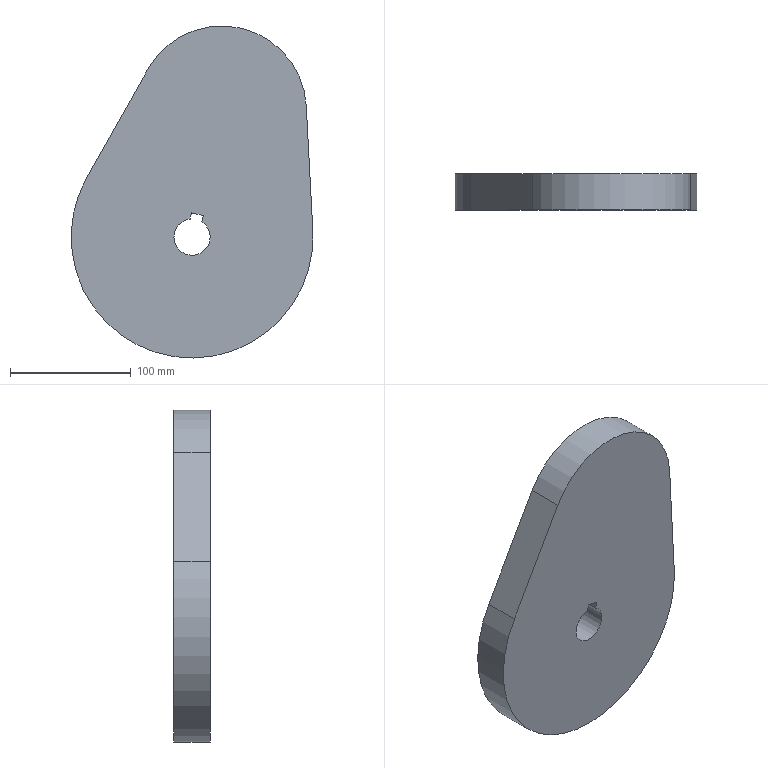Component | NX | CAM | 1 solid | 10 faces | box 200 x 30 x 274.65 mm | volume 1249246 mm3 | plane 7 | cylinder 3 | commonest cylinder face diameters 30 x1 200 x1 140 x1
STEP:
#1=CARTESIAN_POINT('',(0.,0.,0.));
#2=DIRECTION('',(0.,0.,1.));
#3=DIRECTION('',(1.,0.,0.));
#4=AXIS2_PLACEMENT_3D('',#1,#2,#3);
#5=CARTESIAN_POINT('',(298.366,15.,104.911));
#6=VERTEX_POINT('',#5);
#7=CARTESIAN_POINT('',(298.366,-15.,104.911));
#8=VERTEX_POINT('',#7);
#9=CARTESIAN_POINT('',(298.366,15.,104.911));
#10=DIRECTION('',(0.,-1.,0.));
#11=VECTOR('',#10,1.);
#12=LINE('',#9,#11);
#13=CARTESIAN_POINT('',(300.,15.,90.));
#14=DIRECTION('',(0.,-1.,0.));
#15=DIRECTION('',(-0.2286,0.,-0.9735));
#16=AXIS2_PLACEMENT_3D('',#13,#14,#15);
#17=CYLINDRICAL_SURFACE('',#16,15.);
#18=CARTESIAN_POINT('',(3.481,0.));
#19=DIRECTION('',(0.,1.));
#20=VECTOR('',#19,1.);
#21=LINE('',#18,#20);
#22=(GEOMETRIC_REPRESENTATION_CONTEXT(2)PARAMETRIC_REPRESENTATION_CONTEXT()REPRESENTATION_CONTEXT('',''));
#23=DEFINITIONAL_REPRESENTATION('',(#21),#22);
#24=PCURVE('',#17,#23);
#25=CARTESIAN_POINT('',(299.59,15.,110.127));
#26=DIRECTION('',(-0.9735,0.,0.2286));
#27=DIRECTION('',(0.2286,0.,0.9735));
#28=AXIS2_PLACEMENT_3D('',#25,#26,#27);
#29=PLANE('',#28);
#30=CARTESIAN_POINT('',(-5.358,0.));
#31=DIRECTION('',(0.,-1.));
#32=VECTOR('',#31,1.);
#33=LINE('',#30,#32);
#34=(GEOMETRIC_REPRESENTATION_CONTEXT(2)PARAMETRIC_REPRESENTATION_CONTEXT()REPRESENTATION_CONTEXT('',''));
#35=DEFINITIONAL_REPRESENTATION('',(#33),#34);
#36=PCURVE('',#29,#35);
#37=SURFACE_CURVE('',#12,(#24,#36),.PCURVE_S1.);
#38=EDGE_CURVE('',#6,#8,#37,.T.);
#39=ORIENTED_EDGE('',*,*,#38,.F.);
#40=CARTESIAN_POINT('',(308.101,15.,102.625));
#41=VERTEX_POINT('',#40);
#42=CARTESIAN_POINT('',(300.,15.,90.));
#43=DIRECTION('',(0.,-1.,0.));
#44=DIRECTION('',(0.2286,0.,0.9735));
#45=AXIS2_PLACEMENT_3D('',#42,#43,#44);
#46=CIRCLE('',#45,15.);
#47=CARTESIAN_POINT('',(3.142,0.));
#48=DIRECTION('',(1.,0.));
#49=VECTOR('',#48,1.);
#50=LINE('',#47,#49);
#51=(GEOMETRIC_REPRESENTATION_CONTEXT(2)PARAMETRIC_REPRESENTATION_CONTEXT()REPRESENTATION_CONTEXT('',''));
#52=DEFINITIONAL_REPRESENTATION('',(#50),#51);
#53=PCURVE('',#17,#52);
#54=CARTESIAN_POINT('',(300.,15.,90.));
#55=DIRECTION('',(0.,1.,0.));
#56=DIRECTION('',(0.2286,0.,0.9735));
#57=AXIS2_PLACEMENT_3D('',#54,#55,#56);
#58=PLANE('',#57);
#59=CARTESIAN_POINT('',(15.,0.));
#60=CARTESIAN_POINT('',(15.,-25.981));
#61=CARTESIAN_POINT('',(-7.5,-12.99));
#62=CARTESIAN_POINT('',(-30.,-0.));
#63=CARTESIAN_POINT('',(-7.5,12.99));
#64=CARTESIAN_POINT('',(15.,25.981));
#65=CARTESIAN_POINT('',(15.,0.));
#66=(BOUNDED_CURVE()B_SPLINE_CURVE(2,(#59,#60,#61,#62,#63,#64,#65),.UNSPECIFIED.,.T.,.F.)B_SPLINE_CURVE_WITH_KNOTS((1,2,2,2,2,1),(-2.094,0.,2.094,4.189,6.283,8.378),.UNSPECIFIED.)CURVE()GEOMETRIC_REPRESENTATION_ITEM()RATIONAL_B_SPLINE_CURVE((1.,0.5,1.,0.5,1.,0.5,1.))REPRESENTATION_ITEM(''));
#67=(GEOMETRIC_REPRESENTATION_CONTEXT(2)PARAMETRIC_REPRESENTATION_CONTEXT()REPRESENTATION_CONTEXT('',''));
#68=DEFINITIONAL_REPRESENTATION('',(#66),#67);
#69=PCURVE('',#58,#68);
#70=SURFACE_CURVE('',#46,(#53,#69),.PCURVE_S1.);
#71=EDGE_CURVE('',#6,#41,#70,.T.);
#72=ORIENTED_EDGE('',*,*,#71,.T.);
#73=CARTESIAN_POINT('',(308.101,-15.,102.625));
#74=VERTEX_POINT('',#73);
#75=CARTESIAN_POINT('',(308.101,15.,102.625));
#76=DIRECTION('',(0.,-1.,0.));
#77=VECTOR('',#76,1.);
#78=LINE('',#75,#77);
#79=CARTESIAN_POINT('',(9.085,0.));
#80=DIRECTION('',(0.,1.));
#81=VECTOR('',#80,1.);
#82=LINE('',#79,#81);
#83=(GEOMETRIC_REPRESENTATION_CONTEXT(2)PARAMETRIC_REPRESENTATION_CONTEXT()REPRESENTATION_CONTEXT('',''));
#84=DEFINITIONAL_REPRESENTATION('',(#82),#83);
#85=PCURVE('',#17,#84);
#86=CARTESIAN_POINT('',(308.101,15.,102.625));
#87=DIRECTION('',(0.9735,0.,-0.2286));
#88=DIRECTION('',(-0.2286,0.,-0.9735));
#89=AXIS2_PLACEMENT_3D('',#86,#87,#88);
#90=PLANE('',#89);
#91=CARTESIAN_POINT('',(-0.,0.));
#92=DIRECTION('',(0.,-1.));
#93=VECTOR('',#92,1.);
#94=LINE('',#91,#93);
#95=(GEOMETRIC_REPRESENTATION_CONTEXT(2)PARAMETRIC_REPRESENTATION_CONTEXT()REPRESENTATION_CONTEXT('',''));
#96=DEFINITIONAL_REPRESENTATION('',(#94),#95);
#97=PCURVE('',#90,#96);
#98=SURFACE_CURVE('',#78,(#85,#97),.PCURVE_S1.);
#99=EDGE_CURVE('',#41,#74,#98,.T.);
#100=ORIENTED_EDGE('',*,*,#99,.T.);
#101=CARTESIAN_POINT('',(300.,-15.,90.));
#102=DIRECTION('',(0.,-1.,0.));
#103=DIRECTION('',(0.2286,0.,0.9735));
#104=AXIS2_PLACEMENT_3D('',#101,#102,#103);
#105=CIRCLE('',#104,15.);
#106=CARTESIAN_POINT('',(3.142,30.));
#107=DIRECTION('',(1.,0.));
#108=VECTOR('',#107,1.);
#109=LINE('',#106,#108);
#110=(GEOMETRIC_REPRESENTATION_CONTEXT(2)PARAMETRIC_REPRESENTATION_CONTEXT()REPRESENTATION_CONTEXT('',''));
#111=DEFINITIONAL_REPRESENTATION('',(#109),#110);
#112=PCURVE('',#17,#111);
#113=CARTESIAN_POINT('',(300.,-15.,90.));
#114=DIRECTION('',(0.,1.,0.));
#115=DIRECTION('',(0.2286,0.,0.9735));
#116=AXIS2_PLACEMENT_3D('',#113,#114,#115);
#117=PLANE('',#116);
#118=CARTESIAN_POINT('',(15.,0.));
#119=CARTESIAN_POINT('',(15.,-25.981));
#120=CARTESIAN_POINT('',(-7.5,-12.99));
#121=CARTESIAN_POINT('',(-30.,-0.));
#122=CARTESIAN_POINT('',(-7.5,12.99));
#123=CARTESIAN_POINT('',(15.,25.981));
#124=CARTESIAN_POINT('',(15.,0.));
#125=(BOUNDED_CURVE()B_SPLINE_CURVE(2,(#118,#119,#120,#121,#122,#123,#124),.UNSPECIFIED.,.T.,.F.)B_SPLINE_CURVE_WITH_KNOTS((1,2,2,2,2,1),(-2.094,0.,2.094,4.189,6.283,8.378),.UNSPECIFIED.)CURVE()GEOMETRIC_REPRESENTATION_ITEM()RATIONAL_B_SPLINE_CURVE((1.,0.5,1.,0.5,1.,0.5,1.))REPRESENTATION_ITEM(''));
#126=(GEOMETRIC_REPRESENTATION_CONTEXT(2)PARAMETRIC_REPRESENTATION_CONTEXT()REPRESENTATION_CONTEXT('',''));
#127=DEFINITIONAL_REPRESENTATION('',(#125),#126);
#128=PCURVE('',#117,#127);
#129=SURFACE_CURVE('',#105,(#112,#128),.PCURVE_S1.);
#130=EDGE_CURVE('',#8,#74,#129,.T.);
#131=ORIENTED_EDGE('',*,*,#130,.F.);
#132=EDGE_LOOP('',(#39,#72,#100,#131));
#133=FACE_BOUND('',#132,.F.);
#134=ADVANCED_FACE('',(#133),#17,.F.);
#135=CARTESIAN_POINT('',(309.326,-15.,107.84));
#136=VERTEX_POINT('',#135);
#137=CARTESIAN_POINT('',(308.101,-15.,102.625));
#138=DIRECTION('',(0.2286,0.,0.9735));
#139=VECTOR('',#138,1.);
#140=LINE('',#137,#139);
#141=CARTESIAN_POINT('',(0.,-30.));
#142=DIRECTION('',(-1.,0.));
#143=VECTOR('',#142,1.);
#144=LINE('',#141,#143);
#145=(GEOMETRIC_REPRESENTATION_CONTEXT(2)PARAMETRIC_REPRESENTATION_CONTEXT()REPRESENTATION_CONTEXT('',''));
#146=DEFINITIONAL_REPRESENTATION('',(#144),#145);
#147=PCURVE('',#90,#146);
#148=CARTESIAN_POINT('',(14.142,5.));
#149=DIRECTION('',(1.,0.));
#150=VECTOR('',#149,1.);
#151=LINE('',#148,#150);
#152=(GEOMETRIC_REPRESENTATION_CONTEXT(2)PARAMETRIC_REPRESENTATION_CONTEXT()REPRESENTATION_CONTEXT('',''));
#153=DEFINITIONAL_REPRESENTATION('',(#151),#152);
#154=PCURVE('',#117,#153);
#155=SURFACE_CURVE('',#140,(#147,#154),.PCURVE_S1.);
#156=EDGE_CURVE('',#74,#136,#155,.T.);
#157=ORIENTED_EDGE('',*,*,#156,.T.);
#158=CARTESIAN_POINT('',(309.326,15.,107.84));
#159=VERTEX_POINT('',#158);
#160=CARTESIAN_POINT('',(309.326,15.,107.84));
#161=DIRECTION('',(0.,-1.,0.));
#162=VECTOR('',#161,1.);
#163=LINE('',#160,#162);
#164=CARTESIAN_POINT('',(-5.358,0.));
#165=DIRECTION('',(0.,-1.));
#166=VECTOR('',#165,1.);
#167=LINE('',#164,#166);
#168=(GEOMETRIC_REPRESENTATION_CONTEXT(2)PARAMETRIC_REPRESENTATION_CONTEXT()REPRESENTATION_CONTEXT('',''));
#169=DEFINITIONAL_REPRESENTATION('',(#167),#168);
#170=PCURVE('',#90,#169);
#171=CARTESIAN_POINT('',(309.326,15.,107.84));
#172=DIRECTION('',(0.2286,0.,0.9735));
#173=DIRECTION('',(0.9735,0.,-0.2286));
#174=AXIS2_PLACEMENT_3D('',#171,#172,#173);
#175=PLANE('',#174);
#176=CARTESIAN_POINT('',(0.,0.));
#177=DIRECTION('',(0.,-1.));
#178=VECTOR('',#177,1.);
#179=LINE('',#176,#178);
#180=(GEOMETRIC_REPRESENTATION_CONTEXT(2)PARAMETRIC_REPRESENTATION_CONTEXT()REPRESENTATION_CONTEXT('',''));
#181=DEFINITIONAL_REPRESENTATION('',(#179),#180);
#182=PCURVE('',#175,#181);
#183=SURFACE_CURVE('',#163,(#170,#182),.PCURVE_S1.);
#184=EDGE_CURVE('',#159,#136,#183,.T.);
#185=ORIENTED_EDGE('',*,*,#184,.F.);
#186=CARTESIAN_POINT('',(308.101,15.,102.625));
#187=DIRECTION('',(0.2286,0.,0.9735));
#188=VECTOR('',#187,1.);
#189=LINE('',#186,#188);
#190=CARTESIAN_POINT('',(0.,0.));
#191=DIRECTION('',(-1.,0.));
#192=VECTOR('',#191,1.);
#193=LINE('',#190,#192);
#194=(GEOMETRIC_REPRESENTATION_CONTEXT(2)PARAMETRIC_REPRESENTATION_CONTEXT()REPRESENTATION_CONTEXT('',''));
#195=DEFINITIONAL_REPRESENTATION('',(#193),#194);
#196=PCURVE('',#90,#195);
#197=CARTESIAN_POINT('',(14.142,5.));
#198=DIRECTION('',(1.,0.));
#199=VECTOR('',#198,1.);
#200=LINE('',#197,#199);
#201=(GEOMETRIC_REPRESENTATION_CONTEXT(2)PARAMETRIC_REPRESENTATION_CONTEXT()REPRESENTATION_CONTEXT('',''));
#202=DEFINITIONAL_REPRESENTATION('',(#200),#201);
#203=PCURVE('',#58,#202);
#204=SURFACE_CURVE('',#189,(#196,#203),.PCURVE_S1.);
#205=EDGE_CURVE('',#41,#159,#204,.T.);
#206=ORIENTED_EDGE('',*,*,#205,.F.);
#207=ORIENTED_EDGE('',*,*,#99,.T.);
#208=EDGE_LOOP('',(#157,#185,#206,#207));
#209=FACE_BOUND('',#208,.T.);
#210=ADVANCED_FACE('',(#209),#90,.F.);
#211=CARTESIAN_POINT('',(299.59,-15.,110.127));
#212=VERTEX_POINT('',#211);
#213=CARTESIAN_POINT('',(309.326,-15.,107.84));
#214=DIRECTION('',(-0.9735,0.,0.2286));
#215=VECTOR('',#214,1.);
#216=LINE('',#213,#215);
#217=CARTESIAN_POINT('',(0.,-30.));
#218=DIRECTION('',(-1.,0.));
#219=VECTOR('',#218,1.);
#220=LINE('',#217,#219);
#221=(GEOMETRIC_REPRESENTATION_CONTEXT(2)PARAMETRIC_REPRESENTATION_CONTEXT()REPRESENTATION_CONTEXT('',''));
#222=DEFINITIONAL_REPRESENTATION('',(#220),#221);
#223=PCURVE('',#175,#222);
#224=CARTESIAN_POINT('',(19.5,5.));
#225=DIRECTION('',(0.,-1.));
#226=VECTOR('',#225,1.);
#227=LINE('',#224,#226);
#228=(GEOMETRIC_REPRESENTATION_CONTEXT(2)PARAMETRIC_REPRESENTATION_CONTEXT()REPRESENTATION_CONTEXT('',''));
#229=DEFINITIONAL_REPRESENTATION('',(#227),#228);
#230=PCURVE('',#117,#229);
#231=SURFACE_CURVE('',#216,(#223,#230),.PCURVE_S1.);
#232=EDGE_CURVE('',#136,#212,#231,.T.);
#233=ORIENTED_EDGE('',*,*,#232,.T.);
#234=CARTESIAN_POINT('',(299.59,15.,110.127));
#235=VERTEX_POINT('',#234);
#236=CARTESIAN_POINT('',(299.59,15.,110.127));
#237=DIRECTION('',(0.,-1.,0.));
#238=VECTOR('',#237,1.);
#239=LINE('',#236,#238);
#240=CARTESIAN_POINT('',(-10.,0.));
#241=DIRECTION('',(0.,-1.));
#242=VECTOR('',#241,1.);
#243=LINE('',#240,#242);
#244=(GEOMETRIC_REPRESENTATION_CONTEXT(2)PARAMETRIC_REPRESENTATION_CONTEXT()REPRESENTATION_CONTEXT('',''));
#245=DEFINITIONAL_REPRESENTATION('',(#243),#244);
#246=PCURVE('',#175,#245);
#247=CARTESIAN_POINT('',(0.,0.));
#248=DIRECTION('',(0.,-1.));
#249=VECTOR('',#248,1.);
#250=LINE('',#247,#249);
#251=(GEOMETRIC_REPRESENTATION_CONTEXT(2)PARAMETRIC_REPRESENTATION_CONTEXT()REPRESENTATION_CONTEXT('',''));
#252=DEFINITIONAL_REPRESENTATION('',(#250),#251);
#253=PCURVE('',#29,#252);
#254=SURFACE_CURVE('',#239,(#246,#253),.PCURVE_S1.);
#255=EDGE_CURVE('',#235,#212,#254,.T.);
#256=ORIENTED_EDGE('',*,*,#255,.F.);
#257=CARTESIAN_POINT('',(309.326,15.,107.84));
#258=DIRECTION('',(-0.9735,0.,0.2286));
#259=VECTOR('',#258,1.);
#260=LINE('',#257,#259);
#261=CARTESIAN_POINT('',(0.,0.));
#262=DIRECTION('',(-1.,0.));
#263=VECTOR('',#262,1.);
#264=LINE('',#261,#263);
#265=(GEOMETRIC_REPRESENTATION_CONTEXT(2)PARAMETRIC_REPRESENTATION_CONTEXT()REPRESENTATION_CONTEXT('',''));
#266=DEFINITIONAL_REPRESENTATION('',(#264),#265);
#267=PCURVE('',#175,#266);
#268=CARTESIAN_POINT('',(19.5,5.));
#269=DIRECTION('',(0.,-1.));
#270=VECTOR('',#269,1.);
#271=LINE('',#268,#270);
#272=(GEOMETRIC_REPRESENTATION_CONTEXT(2)PARAMETRIC_REPRESENTATION_CONTEXT()REPRESENTATION_CONTEXT('',''));
#273=DEFINITIONAL_REPRESENTATION('',(#271),#272);
#274=PCURVE('',#58,#273);
#275=SURFACE_CURVE('',#260,(#267,#274),.PCURVE_S1.);
#276=EDGE_CURVE('',#159,#235,#275,.T.);
#277=ORIENTED_EDGE('',*,*,#276,.F.);
#278=ORIENTED_EDGE('',*,*,#184,.T.);
#279=EDGE_LOOP('',(#233,#256,#277,#278));
#280=FACE_BOUND('',#279,.T.);
#281=ADVANCED_FACE('',(#280),#175,.F.);
#282=CARTESIAN_POINT('',(399.864,-15.,95.214));
#283=VERTEX_POINT('',#282);
#284=CARTESIAN_POINT('',(212.896,-15.,139.121));
#285=VERTEX_POINT('',#284);
#286=CARTESIAN_POINT('',(300.,-15.,90.));
#287=DIRECTION('',(0.,1.,0.));
#288=DIRECTION('',(0.2286,0.,0.9735));
#289=AXIS2_PLACEMENT_3D('',#286,#287,#288);
#290=CIRCLE('',#289,100.);
#291=CARTESIAN_POINT('',(300.,15.,90.));
#292=DIRECTION('',(0.,-1.,0.));
#293=DIRECTION('',(-0.2286,0.,-0.9735));
#294=AXIS2_PLACEMENT_3D('',#291,#292,#293);
#295=CYLINDRICAL_SURFACE('',#294,100.);
#296=CARTESIAN_POINT('',(3.142,30.));
#297=DIRECTION('',(-1.,0.));
#298=VECTOR('',#297,1.);
#299=LINE('',#296,#298);
#300=(GEOMETRIC_REPRESENTATION_CONTEXT(2)PARAMETRIC_REPRESENTATION_CONTEXT()REPRESENTATION_CONTEXT('',''));
#301=DEFINITIONAL_REPRESENTATION('',(#299),#300);
#302=PCURVE('',#295,#301);
#303=CARTESIAN_POINT('',(0.,0.));
#304=DIRECTION('',(1.,0.));
#305=AXIS2_PLACEMENT_2D('',#303,#304);
#306=CIRCLE('',#305,100.);
#307=(GEOMETRIC_REPRESENTATION_CONTEXT(2)PARAMETRIC_REPRESENTATION_CONTEXT()REPRESENTATION_CONTEXT('',''));
#308=DEFINITIONAL_REPRESENTATION('',(#306),#307);
#309=PCURVE('',#117,#308);
#310=SURFACE_CURVE('',#290,(#302,#309),.PCURVE_S1.);
#311=EDGE_CURVE('',#283,#285,#310,.T.);
#312=ORIENTED_EDGE('',*,*,#311,.T.);
#313=CARTESIAN_POINT('',(212.896,15.,139.121));
#314=VERTEX_POINT('',#313);
#315=CARTESIAN_POINT('',(212.896,15.,139.121));
#316=DIRECTION('',(0.,-1.,0.));
#317=VECTOR('',#316,1.);
#318=LINE('',#315,#317);
#319=CARTESIAN_POINT('',(-1.854,0.));
#320=DIRECTION('',(0.,1.));
#321=VECTOR('',#320,1.);
#322=LINE('',#319,#321);
#323=(GEOMETRIC_REPRESENTATION_CONTEXT(2)PARAMETRIC_REPRESENTATION_CONTEXT()REPRESENTATION_CONTEXT('',''));
#324=DEFINITIONAL_REPRESENTATION('',(#322),#323);
#325=PCURVE('',#295,#324);
#326=CARTESIAN_POINT('',(212.896,15.,139.121));
#327=DIRECTION('',(0.871,0.,-0.4912));
#328=DIRECTION('',(-0.4912,0.,-0.871));
#329=AXIS2_PLACEMENT_3D('',#326,#327,#328);
#330=PLANE('',#329);
#331=CARTESIAN_POINT('',(0.,0.));
#332=DIRECTION('',(0.,-1.));
#333=VECTOR('',#332,1.);
#334=LINE('',#331,#333);
#335=(GEOMETRIC_REPRESENTATION_CONTEXT(2)PARAMETRIC_REPRESENTATION_CONTEXT()REPRESENTATION_CONTEXT('',''));
#336=DEFINITIONAL_REPRESENTATION('',(#334),#335);
#337=PCURVE('',#330,#336);
#338=SURFACE_CURVE('',#318,(#325,#337),.PCURVE_S1.);
#339=EDGE_CURVE('',#314,#285,#338,.T.);
#340=ORIENTED_EDGE('',*,*,#339,.F.);
#341=CARTESIAN_POINT('',(399.864,15.,95.214));
#342=VERTEX_POINT('',#341);
#343=CARTESIAN_POINT('',(300.,15.,90.));
#344=DIRECTION('',(0.,1.,0.));
#345=DIRECTION('',(0.2286,0.,0.9735));
#346=AXIS2_PLACEMENT_3D('',#343,#344,#345);
#347=CIRCLE('',#346,100.);
#348=CARTESIAN_POINT('',(3.142,0.));
#349=DIRECTION('',(-1.,0.));
#350=VECTOR('',#349,1.);
#351=LINE('',#348,#350);
#352=(GEOMETRIC_REPRESENTATION_CONTEXT(2)PARAMETRIC_REPRESENTATION_CONTEXT()REPRESENTATION_CONTEXT('',''));
#353=DEFINITIONAL_REPRESENTATION('',(#351),#352);
#354=PCURVE('',#295,#353);
#355=CARTESIAN_POINT('',(0.,0.));
#356=DIRECTION('',(1.,0.));
#357=AXIS2_PLACEMENT_2D('',#355,#356);
#358=CIRCLE('',#357,100.);
#359=(GEOMETRIC_REPRESENTATION_CONTEXT(2)PARAMETRIC_REPRESENTATION_CONTEXT()REPRESENTATION_CONTEXT('',''));
#360=DEFINITIONAL_REPRESENTATION('',(#358),#359);
#361=PCURVE('',#58,#360);
#362=SURFACE_CURVE('',#347,(#354,#361),.PCURVE_S1.);
#363=EDGE_CURVE('',#342,#314,#362,.T.);
#364=ORIENTED_EDGE('',*,*,#363,.F.);
#365=CARTESIAN_POINT('',(399.864,15.,95.214));
#366=DIRECTION('',(0.,-1.,0.));
#367=VECTOR('',#366,1.);
#368=LINE('',#365,#367);
#369=CARTESIAN_POINT('',(1.854,0.));
#370=DIRECTION('',(0.,1.));
#371=VECTOR('',#370,1.);
#372=LINE('',#369,#371);
#373=(GEOMETRIC_REPRESENTATION_CONTEXT(2)PARAMETRIC_REPRESENTATION_CONTEXT()REPRESENTATION_CONTEXT('',''));
#374=DEFINITIONAL_REPRESENTATION('',(#372),#373);
#375=PCURVE('',#295,#374);
#376=CARTESIAN_POINT('',(394.481,15.,198.303));
#377=DIRECTION('',(-0.9986,0.,-0.05214));
#378=DIRECTION('',(-0.05214,0.,0.9986));
#379=AXIS2_PLACEMENT_3D('',#376,#377,#378);
#380=PLANE('',#379);
#381=CARTESIAN_POINT('',(-103.229,0.));
#382=DIRECTION('',(0.,-1.));
#383=VECTOR('',#382,1.);
#384=LINE('',#381,#383);
#385=(GEOMETRIC_REPRESENTATION_CONTEXT(2)PARAMETRIC_REPRESENTATION_CONTEXT()REPRESENTATION_CONTEXT('',''));
#386=DEFINITIONAL_REPRESENTATION('',(#384),#385);
#387=PCURVE('',#380,#386);
#388=SURFACE_CURVE('',#368,(#375,#387),.PCURVE_S1.);
#389=EDGE_CURVE('',#342,#283,#388,.T.);
#390=ORIENTED_EDGE('',*,*,#389,.T.);
#391=EDGE_LOOP('',(#312,#340,#364,#390));
#392=FACE_BOUND('',#391,.T.);
#393=ADVANCED_FACE('',(#392),#295,.T.);
#394=CARTESIAN_POINT('',(263.604,-15.,229.038));
#395=VERTEX_POINT('',#394);
#396=CARTESIAN_POINT('',(212.896,-15.,139.121));
#397=DIRECTION('',(0.4912,0.,0.871));
#398=VECTOR('',#397,1.);
#399=LINE('',#396,#398);
#400=CARTESIAN_POINT('',(0.,-30.));
#401=DIRECTION('',(-1.,0.));
#402=VECTOR('',#401,1.);
#403=LINE('',#400,#402);
#404=(GEOMETRIC_REPRESENTATION_CONTEXT(2)PARAMETRIC_REPRESENTATION_CONTEXT()REPRESENTATION_CONTEXT('',''));
#405=DEFINITIONAL_REPRESENTATION('',(#403),#404);
#406=PCURVE('',#330,#405);
#407=CARTESIAN_POINT('',(27.907,-96.027));
#408=DIRECTION('',(0.9603,0.2791));
#409=VECTOR('',#408,1.);
#410=LINE('',#407,#409);
#411=(GEOMETRIC_REPRESENTATION_CONTEXT(2)PARAMETRIC_REPRESENTATION_CONTEXT()REPRESENTATION_CONTEXT('',''));
#412=DEFINITIONAL_REPRESENTATION('',(#410),#411);
#413=PCURVE('',#117,#412);
#414=SURFACE_CURVE('',#399,(#406,#413),.PCURVE_S1.);
#415=EDGE_CURVE('',#285,#395,#414,.T.);
#416=ORIENTED_EDGE('',*,*,#415,.T.);
#417=CARTESIAN_POINT('',(263.604,15.,229.038));
#418=VERTEX_POINT('',#417);
#419=CARTESIAN_POINT('',(263.604,15.,229.038));
#420=DIRECTION('',(0.,-1.,0.));
#421=VECTOR('',#420,1.);
#422=LINE('',#419,#421);
#423=CARTESIAN_POINT('',(-103.229,0.));
#424=DIRECTION('',(0.,-1.));
#425=VECTOR('',#424,1.);
#426=LINE('',#423,#425);
#427=(GEOMETRIC_REPRESENTATION_CONTEXT(2)PARAMETRIC_REPRESENTATION_CONTEXT()REPRESENTATION_CONTEXT('',''));
#428=DEFINITIONAL_REPRESENTATION('',(#426),#427);
#429=PCURVE('',#330,#428);
#430=CARTESIAN_POINT('',(324.576,15.,194.653));
#431=DIRECTION('',(0.,-1.,0.));
#432=DIRECTION('',(-0.2286,0.,-0.9735));
#433=AXIS2_PLACEMENT_3D('',#430,#431,#432);
#434=CYLINDRICAL_SURFACE('',#433,70.);
#435=CARTESIAN_POINT('',(4.43,0.));
#436=DIRECTION('',(0.,1.));
#437=VECTOR('',#436,1.);
#438=LINE('',#435,#437);
#439=(GEOMETRIC_REPRESENTATION_CONTEXT(2)PARAMETRIC_REPRESENTATION_CONTEXT()REPRESENTATION_CONTEXT('',''));
#440=DEFINITIONAL_REPRESENTATION('',(#438),#439);
#441=PCURVE('',#434,#440);
#442=SURFACE_CURVE('',#422,(#429,#441),.PCURVE_S1.);
#443=EDGE_CURVE('',#418,#395,#442,.T.);
#444=ORIENTED_EDGE('',*,*,#443,.F.);
#445=CARTESIAN_POINT('',(212.896,15.,139.121));
#446=DIRECTION('',(0.4912,0.,0.871));
#447=VECTOR('',#446,1.);
#448=LINE('',#445,#447);
#449=CARTESIAN_POINT('',(0.,0.));
#450=DIRECTION('',(-1.,0.));
#451=VECTOR('',#450,1.);
#452=LINE('',#449,#451);
#453=(GEOMETRIC_REPRESENTATION_CONTEXT(2)PARAMETRIC_REPRESENTATION_CONTEXT()REPRESENTATION_CONTEXT('',''));
#454=DEFINITIONAL_REPRESENTATION('',(#452),#453);
#455=PCURVE('',#330,#454);
#456=CARTESIAN_POINT('',(27.907,-96.027));
#457=DIRECTION('',(0.9603,0.2791));
#458=VECTOR('',#457,1.);
#459=LINE('',#456,#458);
#460=(GEOMETRIC_REPRESENTATION_CONTEXT(2)PARAMETRIC_REPRESENTATION_CONTEXT()REPRESENTATION_CONTEXT('',''));
#461=DEFINITIONAL_REPRESENTATION('',(#459),#460);
#462=PCURVE('',#58,#461);
#463=SURFACE_CURVE('',#448,(#455,#462),.PCURVE_S1.);
#464=EDGE_CURVE('',#314,#418,#463,.T.);
#465=ORIENTED_EDGE('',*,*,#464,.F.);
#466=ORIENTED_EDGE('',*,*,#339,.T.);
#467=EDGE_LOOP('',(#416,#444,#465,#466));
#468=FACE_BOUND('',#467,.T.);
#469=ADVANCED_FACE('',(#468),#330,.F.);
#470=CARTESIAN_POINT('',(394.481,-15.,198.303));
#471=VERTEX_POINT('',#470);
#472=CARTESIAN_POINT('',(324.576,-15.,194.653));
#473=DIRECTION('',(0.,1.,0.));
#474=DIRECTION('',(0.2286,0.,0.9735));
#475=AXIS2_PLACEMENT_3D('',#472,#473,#474);
#476=CIRCLE('',#475,70.);
#477=CARTESIAN_POINT('',(9.425,30.));
#478=DIRECTION('',(-1.,0.));
#479=VECTOR('',#478,1.);
#480=LINE('',#477,#479);
#481=(GEOMETRIC_REPRESENTATION_CONTEXT(2)PARAMETRIC_REPRESENTATION_CONTEXT()REPRESENTATION_CONTEXT('',''));
#482=DEFINITIONAL_REPRESENTATION('',(#480),#481);
#483=PCURVE('',#434,#482);
#484=CARTESIAN_POINT('',(107.5,0.));
#485=DIRECTION('',(1.,0.));
#486=AXIS2_PLACEMENT_2D('',#484,#485);
#487=CIRCLE('',#486,70.);
#488=(GEOMETRIC_REPRESENTATION_CONTEXT(2)PARAMETRIC_REPRESENTATION_CONTEXT()REPRESENTATION_CONTEXT('',''));
#489=DEFINITIONAL_REPRESENTATION('',(#487),#488);
#490=PCURVE('',#117,#489);
#491=SURFACE_CURVE('',#476,(#483,#490),.PCURVE_S1.);
#492=EDGE_CURVE('',#395,#471,#491,.T.);
#493=ORIENTED_EDGE('',*,*,#492,.T.);
#494=CARTESIAN_POINT('',(394.481,15.,198.303));
#495=VERTEX_POINT('',#494);
#496=CARTESIAN_POINT('',(394.481,15.,198.303));
#497=DIRECTION('',(0.,-1.,0.));
#498=VECTOR('',#497,1.);
#499=LINE('',#496,#498);
#500=CARTESIAN_POINT('',(1.854,0.));
#501=DIRECTION('',(0.,1.));
#502=VECTOR('',#501,1.);
#503=LINE('',#500,#502);
#504=(GEOMETRIC_REPRESENTATION_CONTEXT(2)PARAMETRIC_REPRESENTATION_CONTEXT()REPRESENTATION_CONTEXT('',''));
#505=DEFINITIONAL_REPRESENTATION('',(#503),#504);
#506=PCURVE('',#434,#505);
#507=CARTESIAN_POINT('',(0.,0.));
#508=DIRECTION('',(0.,-1.));
#509=VECTOR('',#508,1.);
#510=LINE('',#507,#509);
#511=(GEOMETRIC_REPRESENTATION_CONTEXT(2)PARAMETRIC_REPRESENTATION_CONTEXT()REPRESENTATION_CONTEXT('',''));
#512=DEFINITIONAL_REPRESENTATION('',(#510),#511);
#513=PCURVE('',#380,#512);
#514=SURFACE_CURVE('',#499,(#506,#513),.PCURVE_S1.);
#515=EDGE_CURVE('',#495,#471,#514,.T.);
#516=ORIENTED_EDGE('',*,*,#515,.F.);
#517=CARTESIAN_POINT('',(324.576,15.,194.653));
#518=DIRECTION('',(0.,1.,0.));
#519=DIRECTION('',(0.2286,0.,0.9735));
#520=AXIS2_PLACEMENT_3D('',#517,#518,#519);
#521=CIRCLE('',#520,70.);
#522=CARTESIAN_POINT('',(9.425,0.));
#523=DIRECTION('',(-1.,0.));
#524=VECTOR('',#523,1.);
#525=LINE('',#522,#524);
#526=(GEOMETRIC_REPRESENTATION_CONTEXT(2)PARAMETRIC_REPRESENTATION_CONTEXT()REPRESENTATION_CONTEXT('',''));
#527=DEFINITIONAL_REPRESENTATION('',(#525),#526);
#528=PCURVE('',#434,#527);
#529=CARTESIAN_POINT('',(107.5,0.));
#530=DIRECTION('',(1.,0.));
#531=AXIS2_PLACEMENT_2D('',#529,#530);
#532=CIRCLE('',#531,70.);
#533=(GEOMETRIC_REPRESENTATION_CONTEXT(2)PARAMETRIC_REPRESENTATION_CONTEXT()REPRESENTATION_CONTEXT('',''));
#534=DEFINITIONAL_REPRESENTATION('',(#532),#533);
#535=PCURVE('',#58,#534);
#536=SURFACE_CURVE('',#521,(#528,#535),.PCURVE_S1.);
#537=EDGE_CURVE('',#418,#495,#536,.T.);
#538=ORIENTED_EDGE('',*,*,#537,.F.);
#539=ORIENTED_EDGE('',*,*,#443,.T.);
#540=EDGE_LOOP('',(#493,#516,#538,#539));
#541=FACE_BOUND('',#540,.T.);
#542=ADVANCED_FACE('',(#541),#434,.T.);
#543=CARTESIAN_POINT('',(394.481,-15.,198.303));
#544=DIRECTION('',(0.05214,0.,-0.9986));
#545=VECTOR('',#544,1.);
#546=LINE('',#543,#545);
#547=CARTESIAN_POINT('',(0.,-30.));
#548=DIRECTION('',(-1.,0.));
#549=VECTOR('',#548,1.);
#550=LINE('',#547,#549);
#551=(GEOMETRIC_REPRESENTATION_CONTEXT(2)PARAMETRIC_REPRESENTATION_CONTEXT()REPRESENTATION_CONTEXT('',''));
#552=DEFINITIONAL_REPRESENTATION('',(#550),#551);
#553=PCURVE('',#380,#552);
#554=CARTESIAN_POINT('',(127.035,67.219));
#555=DIRECTION('',(-0.9603,0.2791));
#556=VECTOR('',#555,1.);
#557=LINE('',#554,#556);
#558=(GEOMETRIC_REPRESENTATION_CONTEXT(2)PARAMETRIC_REPRESENTATION_CONTEXT()REPRESENTATION_CONTEXT('',''));
#559=DEFINITIONAL_REPRESENTATION('',(#557),#558);
#560=PCURVE('',#117,#559);
#561=SURFACE_CURVE('',#546,(#553,#560),.PCURVE_S1.);
#562=EDGE_CURVE('',#471,#283,#561,.T.);
#563=ORIENTED_EDGE('',*,*,#562,.T.);
#564=ORIENTED_EDGE('',*,*,#389,.F.);
#565=CARTESIAN_POINT('',(394.481,15.,198.303));
#566=DIRECTION('',(0.05214,0.,-0.9986));
#567=VECTOR('',#566,1.);
#568=LINE('',#565,#567);
#569=CARTESIAN_POINT('',(0.,0.));
#570=DIRECTION('',(-1.,0.));
#571=VECTOR('',#570,1.);
#572=LINE('',#569,#571);
#573=(GEOMETRIC_REPRESENTATION_CONTEXT(2)PARAMETRIC_REPRESENTATION_CONTEXT()REPRESENTATION_CONTEXT('',''));
#574=DEFINITIONAL_REPRESENTATION('',(#572),#573);
#575=PCURVE('',#380,#574);
#576=CARTESIAN_POINT('',(127.035,67.219));
#577=DIRECTION('',(-0.9603,0.2791));
#578=VECTOR('',#577,1.);
#579=LINE('',#576,#578);
#580=(GEOMETRIC_REPRESENTATION_CONTEXT(2)PARAMETRIC_REPRESENTATION_CONTEXT()REPRESENTATION_CONTEXT('',''));
#581=DEFINITIONAL_REPRESENTATION('',(#579),#580);
#582=PCURVE('',#58,#581);
#583=SURFACE_CURVE('',#568,(#575,#582),.PCURVE_S1.);
#584=EDGE_CURVE('',#495,#342,#583,.T.);
#585=ORIENTED_EDGE('',*,*,#584,.F.);
#586=ORIENTED_EDGE('',*,*,#515,.T.);
#587=EDGE_LOOP('',(#563,#564,#585,#586));
#588=FACE_BOUND('',#587,.T.);
#589=ADVANCED_FACE('',(#588),#380,.F.);
#590=CARTESIAN_POINT('',(299.59,-15.,110.127));
#591=DIRECTION('',(-0.2286,0.,-0.9735));
#592=VECTOR('',#591,1.);
#593=LINE('',#590,#592);
#594=CARTESIAN_POINT('',(0.,-30.));
#595=DIRECTION('',(-1.,0.));
#596=VECTOR('',#595,1.);
#597=LINE('',#594,#596);
#598=(GEOMETRIC_REPRESENTATION_CONTEXT(2)PARAMETRIC_REPRESENTATION_CONTEXT()REPRESENTATION_CONTEXT('',''));
#599=DEFINITIONAL_REPRESENTATION('',(#597),#598);
#600=PCURVE('',#29,#599);
#601=CARTESIAN_POINT('',(19.5,-5.));
#602=DIRECTION('',(-1.,0.));
#603=VECTOR('',#602,1.);
#604=LINE('',#601,#603);
#605=(GEOMETRIC_REPRESENTATION_CONTEXT(2)PARAMETRIC_REPRESENTATION_CONTEXT()REPRESENTATION_CONTEXT('',''));
#606=DEFINITIONAL_REPRESENTATION('',(#604),#605);
#607=PCURVE('',#117,#606);
#608=SURFACE_CURVE('',#593,(#600,#607),.PCURVE_S1.);
#609=EDGE_CURVE('',#212,#8,#608,.T.);
#610=ORIENTED_EDGE('',*,*,#609,.T.);
#611=ORIENTED_EDGE('',*,*,#38,.F.);
#612=CARTESIAN_POINT('',(299.59,15.,110.127));
#613=DIRECTION('',(-0.2286,0.,-0.9735));
#614=VECTOR('',#613,1.);
#615=LINE('',#612,#614);
#616=CARTESIAN_POINT('',(0.,0.));
#617=DIRECTION('',(-1.,0.));
#618=VECTOR('',#617,1.);
#619=LINE('',#616,#618);
#620=(GEOMETRIC_REPRESENTATION_CONTEXT(2)PARAMETRIC_REPRESENTATION_CONTEXT()REPRESENTATION_CONTEXT('',''));
#621=DEFINITIONAL_REPRESENTATION('',(#619),#620);
#622=PCURVE('',#29,#621);
#623=CARTESIAN_POINT('',(19.5,-5.));
#624=DIRECTION('',(-1.,0.));
#625=VECTOR('',#624,1.);
#626=LINE('',#623,#625);
#627=(GEOMETRIC_REPRESENTATION_CONTEXT(2)PARAMETRIC_REPRESENTATION_CONTEXT()REPRESENTATION_CONTEXT('',''));
#628=DEFINITIONAL_REPRESENTATION('',(#626),#627);
#629=PCURVE('',#58,#628);
#630=SURFACE_CURVE('',#615,(#622,#629),.PCURVE_S1.);
#631=EDGE_CURVE('',#235,#6,#630,.T.);
#632=ORIENTED_EDGE('',*,*,#631,.F.);
#633=ORIENTED_EDGE('',*,*,#255,.T.);
#634=EDGE_LOOP('',(#610,#611,#632,#633));
#635=FACE_BOUND('',#634,.T.);
#636=ADVANCED_FACE('',(#635),#29,.F.);
#637=ORIENTED_EDGE('',*,*,#363,.T.);
#638=ORIENTED_EDGE('',*,*,#464,.T.);
#639=ORIENTED_EDGE('',*,*,#537,.T.);
#640=ORIENTED_EDGE('',*,*,#584,.T.);
#641=EDGE_LOOP('',(#637,#638,#639,#640));
#642=FACE_BOUND('',#641,.T.);
#643=ORIENTED_EDGE('',*,*,#71,.T.);
#644=ORIENTED_EDGE('',*,*,#205,.T.);
#645=ORIENTED_EDGE('',*,*,#276,.T.);
#646=ORIENTED_EDGE('',*,*,#631,.T.);
#647=EDGE_LOOP('',(#643,#644,#645,#646));
#648=FACE_BOUND('',#647,.T.);
#649=ADVANCED_FACE('',(#642,#648),#58,.T.);
#650=ORIENTED_EDGE('',*,*,#311,.F.);
#651=ORIENTED_EDGE('',*,*,#562,.F.);
#652=ORIENTED_EDGE('',*,*,#492,.F.);
#653=ORIENTED_EDGE('',*,*,#415,.F.);
#654=EDGE_LOOP('',(#650,#651,#652,#653));
#655=FACE_BOUND('',#654,.T.);
#656=ORIENTED_EDGE('',*,*,#130,.F.);
#657=ORIENTED_EDGE('',*,*,#609,.F.);
#658=ORIENTED_EDGE('',*,*,#232,.F.);
#659=ORIENTED_EDGE('',*,*,#156,.F.);
#660=EDGE_LOOP('',(#656,#657,#658,#659));
#661=FACE_BOUND('',#660,.T.);
#662=ADVANCED_FACE('',(#655,#661),#117,.F.);
#663=CLOSED_SHELL('',(#134,#210,#281,#393,#469,#542,#589,#636,#649,#662));
#664=MANIFOLD_SOLID_BREP('',#663);
#665=(LENGTH_UNIT()NAMED_UNIT(*)SI_UNIT(.MILLI.,.METRE.));
#666=UNCERTAINTY_MEASURE_WITH_UNIT(LENGTH_MEASURE(0.0000001),#665,'','');
#667=(NAMED_UNIT(*)PLANE_ANGLE_UNIT()SI_UNIT($,.RADIAN.));
#668=(NAMED_UNIT(*)SI_UNIT($,.STERADIAN.)SOLID_ANGLE_UNIT());
#669=(GEOMETRIC_REPRESENTATION_CONTEXT(3)GLOBAL_UNCERTAINTY_ASSIGNED_CONTEXT((#666))GLOBAL_UNIT_ASSIGNED_CONTEXT((#665,#667,#668))REPRESENTATION_CONTEXT('',''));
#670=ADVANCED_BREP_SHAPE_REPRESENTATION('',(#4,#664),#669);